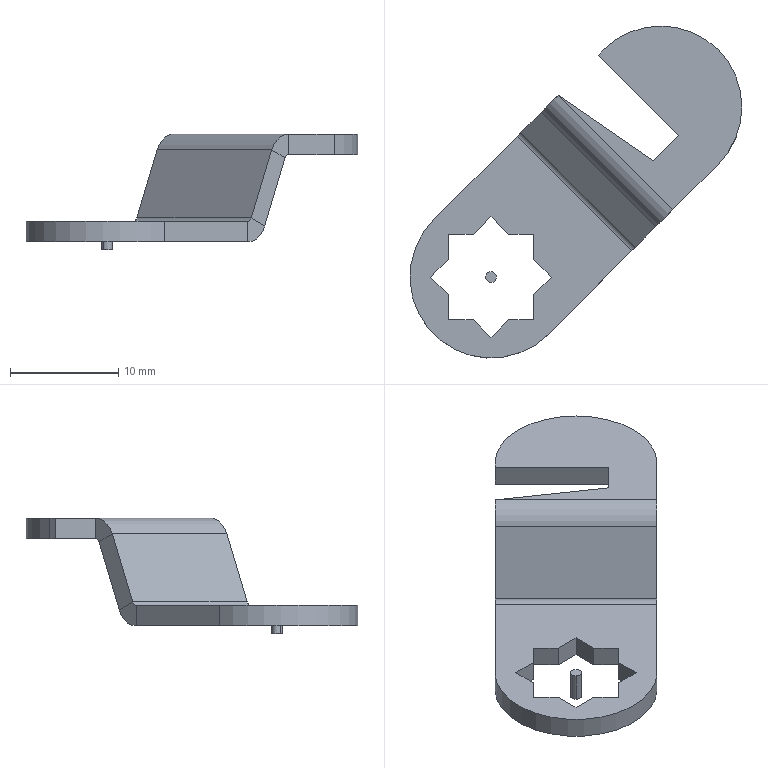Component | SolidWorks | PC-CAJ-P09-1_Lengueta Chapa Guantera Duesco A-1 | 2 solids | 46 faces | volume 882 mm3 | plane 37 | cylinder 9 | commonest cylinder face diameters 1 x4 14.95 x3 4.8 x2 | material Plain Carbon Steel